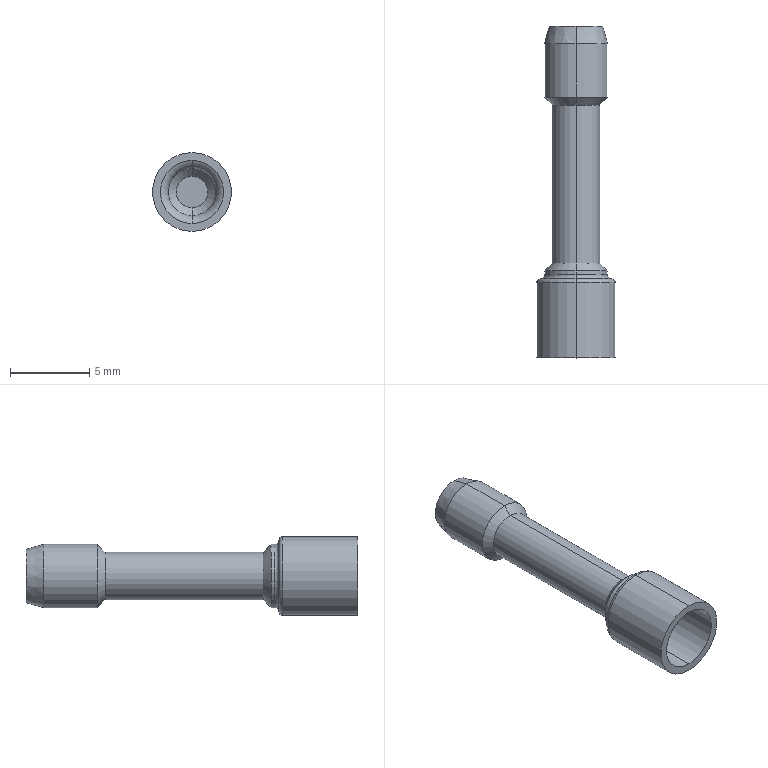Component | SolidWorks | PenTail-1 | 1 solid | 37 faces | box 5 x 21 x 5 mm | volume 112 mm3 | cylinder 16 | cone 12 | torus 6 | plane 3 | commonest cylinder face diameters 3 x6 4 x6 2 x2 5 x2
STEP:
#1=CARTESIAN_POINT('',(-2.232,1.614,-1.121));
#2=VERTEX_POINT('',#1);
#3=CARTESIAN_POINT('',(-2.232,1.614,-1.239));
#4=VERTEX_POINT('',#3);
#5=CARTESIAN_POINT('',(-2.232,1.614,-1.18));
#6=DIRECTION('',(0.,1.,0.));
#7=DIRECTION('',(0.,0.,-1.));
#8=AXIS2_PLACEMENT_3D('',#5,#6,#7);
#9=CIRCLE('',#8,0.05906);
#10=EDGE_CURVE('',#2,#4,#9,.T.);
#11=ORIENTED_EDGE('',*,*,#10,.T.);
#12=CARTESIAN_POINT('',(-2.232,1.586,-1.258));
#13=VERTEX_POINT('',#12);
#14=CARTESIAN_POINT('',(-2.232,1.614,-1.268));
#15=DIRECTION('',(1.,0.,0.));
#16=DIRECTION('',(0.,0.,-1.));
#17=AXIS2_PLACEMENT_3D('',#14,#15,#16);
#18=CIRCLE('',#17,0.02953);
#19=EDGE_CURVE('',#4,#13,#18,.T.);
#20=ORIENTED_EDGE('',*,*,#19,.T.);
#21=CARTESIAN_POINT('',(-2.232,1.586,-1.101));
#22=VERTEX_POINT('',#21);
#23=CARTESIAN_POINT('',(-2.232,1.586,-1.18));
#24=DIRECTION('',(0.,-1.,0.));
#25=DIRECTION('',(0.,0.,1.));
#26=AXIS2_PLACEMENT_3D('',#23,#24,#25);
#27=CIRCLE('',#26,0.07874);
#28=EDGE_CURVE('',#13,#22,#27,.T.);
#29=ORIENTED_EDGE('',*,*,#28,.T.);
#30=CARTESIAN_POINT('',(-2.232,1.614,-1.091));
#31=DIRECTION('',(-1.,0.,0.));
#32=DIRECTION('',(0.,0.,1.));
#33=AXIS2_PLACEMENT_3D('',#30,#31,#32);
#34=CIRCLE('',#33,0.02953);
#35=EDGE_CURVE('',#2,#22,#34,.T.);
#36=ORIENTED_EDGE('',*,*,#35,.F.);
#37=EDGE_LOOP('',(#11,#20,#29,#36));
#38=FACE_OUTER_BOUND('',#37,.T.);
#39=CARTESIAN_POINT('',(-2.232,1.614,-1.18));
#40=DIRECTION('',(0.,1.,0.));
#41=DIRECTION('',(0.,0.,1.));
#42=AXIS2_PLACEMENT_3D('',#39,#40,#41);
#43=TOROIDAL_SURFACE('',#42,0.08858,0.02953);
#44=ADVANCED_FACE('',(#38),#43,.T.);
#45=CARTESIAN_POINT('',(-2.232,2.214,-1.231));
#46=VERTEX_POINT('',#45);
#47=CARTESIAN_POINT('',(-2.232,2.214,-1.128));
#48=VERTEX_POINT('',#47);
#49=CARTESIAN_POINT('',(-2.232,2.214,-1.18));
#50=DIRECTION('',(0.,1.,0.));
#51=DIRECTION('',(0.,0.,1.));
#52=AXIS2_PLACEMENT_3D('',#49,#50,#51);
#53=CIRCLE('',#52,0.05182);
#54=EDGE_CURVE('',#46,#48,#53,.T.);
#55=ORIENTED_EDGE('',*,*,#54,.T.);
#56=CARTESIAN_POINT('',(-2.232,2.187,-1.121));
#57=VERTEX_POINT('',#56);
#58=CARTESIAN_POINT('',(-2.232,2.185,-1.12));
#59=DIRECTION('',(0.,-0.9659,0.2588));
#60=VECTOR('',#59,39.37);
#61=LINE('',#58,#60);
#62=EDGE_CURVE('',#48,#57,#61,.T.);
#63=ORIENTED_EDGE('',*,*,#62,.T.);
#64=CARTESIAN_POINT('',(-2.232,2.187,-1.239));
#65=VERTEX_POINT('',#64);
#66=CARTESIAN_POINT('',(-2.232,2.187,-1.18));
#67=DIRECTION('',(0.,-1.,0.));
#68=DIRECTION('',(0.,0.,-1.));
#69=AXIS2_PLACEMENT_3D('',#66,#67,#68);
#70=CIRCLE('',#69,0.05906);
#71=EDGE_CURVE('',#57,#65,#70,.T.);
#72=ORIENTED_EDGE('',*,*,#71,.T.);
#73=CARTESIAN_POINT('',(-2.232,2.185,-1.239));
#74=DIRECTION('',(0.,-0.9659,-0.2588));
#75=VECTOR('',#74,39.37);
#76=LINE('',#73,#75);
#77=EDGE_CURVE('',#46,#65,#76,.T.);
#78=ORIENTED_EDGE('',*,*,#77,.F.);
#79=EDGE_LOOP('',(#55,#63,#72,#78));
#80=FACE_OUTER_BOUND('',#79,.T.);
#81=CARTESIAN_POINT('',(-2.232,2.185,-1.18));
#82=DIRECTION('',(0.,-1.,0.));
#83=DIRECTION('',(0.,0.,-1.));
#84=AXIS2_PLACEMENT_3D('',#81,#82,#83);
#85=CONICAL_SURFACE('',#84,0.05973,0.2618);
#86=ADVANCED_FACE('',(#80),#85,.F.);
#87=CARTESIAN_POINT('',(-2.232,1.635,-1.14));
#88=VERTEX_POINT('',#87);
#89=CARTESIAN_POINT('',(-2.232,1.635,-1.219));
#90=VERTEX_POINT('',#89);
#91=CARTESIAN_POINT('',(-2.232,1.635,-1.18));
#92=DIRECTION('',(0.,-1.,0.));
#93=DIRECTION('',(0.,0.,-1.));
#94=AXIS2_PLACEMENT_3D('',#91,#92,#93);
#95=CIRCLE('',#94,0.03937);
#96=EDGE_CURVE('',#88,#90,#95,.T.);
#97=ORIENTED_EDGE('',*,*,#96,.F.);
#98=CARTESIAN_POINT('',(-2.232,1.615,-1.121));
#99=VERTEX_POINT('',#98);
#100=CARTESIAN_POINT('',(-2.232,1.61,-1.115));
#101=DIRECTION('',(0.,-0.7071,0.7071));
#102=VECTOR('',#101,39.37);
#103=LINE('',#100,#102);
#104=EDGE_CURVE('',#88,#99,#103,.T.);
#105=ORIENTED_EDGE('',*,*,#104,.T.);
#106=CARTESIAN_POINT('',(-2.232,1.615,-1.239));
#107=VERTEX_POINT('',#106);
#108=CARTESIAN_POINT('',(-2.232,1.615,-1.18));
#109=DIRECTION('',(0.,-1.,0.));
#110=DIRECTION('',(0.,0.,-1.));
#111=AXIS2_PLACEMENT_3D('',#108,#109,#110);
#112=CIRCLE('',#111,0.05906);
#113=EDGE_CURVE('',#99,#107,#112,.T.);
#114=ORIENTED_EDGE('',*,*,#113,.T.);
#115=CARTESIAN_POINT('',(-2.232,1.61,-1.244));
#116=DIRECTION('',(0.,-0.7071,-0.7071));
#117=VECTOR('',#116,39.37);
#118=LINE('',#115,#117);
#119=EDGE_CURVE('',#90,#107,#118,.T.);
#120=ORIENTED_EDGE('',*,*,#119,.F.);
#121=EDGE_LOOP('',(#97,#105,#114,#120));
#122=FACE_OUTER_BOUND('',#121,.T.);
#123=CARTESIAN_POINT('',(-2.232,1.61,-1.18));
#124=DIRECTION('',(0.,-1.,0.));
#125=DIRECTION('',(0.,0.,-1.));
#126=AXIS2_PLACEMENT_3D('',#123,#124,#125);
#127=CONICAL_SURFACE('',#126,0.06482,0.7854);
#128=ADVANCED_FACE('',(#122),#127,.F.);
#129=CARTESIAN_POINT('',(-2.232,2.045,-1.14));
#130=VERTEX_POINT('',#129);
#131=CARTESIAN_POINT('',(-2.232,2.045,-1.219));
#132=VERTEX_POINT('',#131);
#133=CARTESIAN_POINT('',(-2.232,2.045,-1.18));
#134=DIRECTION('',(0.,-1.,0.));
#135=DIRECTION('',(0.,0.,1.));
#136=AXIS2_PLACEMENT_3D('',#133,#134,#135);
#137=CIRCLE('',#136,0.03937);
#138=EDGE_CURVE('',#130,#132,#137,.T.);
#139=ORIENTED_EDGE('',*,*,#138,.T.);
#140=CARTESIAN_POINT('',(-2.232,2.065,-1.239));
#141=VERTEX_POINT('',#140);
#142=CARTESIAN_POINT('',(-2.232,2.051,-1.225));
#143=DIRECTION('',(0.,0.7071,-0.7071));
#144=VECTOR('',#143,39.37);
#145=LINE('',#142,#144);
#146=EDGE_CURVE('',#132,#141,#145,.T.);
#147=ORIENTED_EDGE('',*,*,#146,.T.);
#148=CARTESIAN_POINT('',(-2.232,2.065,-1.121));
#149=VERTEX_POINT('',#148);
#150=CARTESIAN_POINT('',(-2.232,2.065,-1.18));
#151=DIRECTION('',(0.,1.,0.));
#152=DIRECTION('',(0.,0.,1.));
#153=AXIS2_PLACEMENT_3D('',#150,#151,#152);
#154=CIRCLE('',#153,0.05906);
#155=EDGE_CURVE('',#141,#149,#154,.T.);
#156=ORIENTED_EDGE('',*,*,#155,.T.);
#157=CARTESIAN_POINT('',(-2.232,2.051,-1.134));
#158=DIRECTION('',(0.,0.7071,0.7071));
#159=VECTOR('',#158,39.37);
#160=LINE('',#157,#159);
#161=EDGE_CURVE('',#130,#149,#160,.T.);
#162=ORIENTED_EDGE('',*,*,#161,.F.);
#163=EDGE_LOOP('',(#139,#147,#156,#162));
#164=FACE_OUTER_BOUND('',#163,.T.);
#165=CARTESIAN_POINT('',(-2.232,2.051,-1.18));
#166=DIRECTION('',(0.,1.,0.));
#167=DIRECTION('',(0.,0.,1.));
#168=AXIS2_PLACEMENT_3D('',#165,#166,#167);
#169=CONICAL_SURFACE('',#168,0.04514,0.7854);
#170=ADVANCED_FACE('',(#164),#169,.F.);
#171=ORIENTED_EDGE('',*,*,#71,.F.);
#172=CARTESIAN_POINT('',(-2.232,1.407,-1.121));
#173=DIRECTION('',(0.,-1.,0.));
#174=VECTOR('',#173,39.37);
#175=LINE('',#172,#174);
#176=EDGE_CURVE('',#57,#149,#175,.T.);
#177=ORIENTED_EDGE('',*,*,#176,.T.);
#178=ORIENTED_EDGE('',*,*,#155,.F.);
#179=CARTESIAN_POINT('',(-2.232,1.407,-1.239));
#180=DIRECTION('',(0.,-1.,0.));
#181=VECTOR('',#180,39.37);
#182=LINE('',#179,#181);
#183=EDGE_CURVE('',#65,#141,#182,.T.);
#184=ORIENTED_EDGE('',*,*,#183,.F.);
#185=EDGE_LOOP('',(#171,#177,#178,#184));
#186=FACE_OUTER_BOUND('',#185,.T.);
#187=CARTESIAN_POINT('',(-2.232,1.407,-1.18));
#188=DIRECTION('',(0.,-1.,0.));
#189=DIRECTION('',(0.,0.,-1.));
#190=AXIS2_PLACEMENT_3D('',#187,#188,#189);
#191=CYLINDRICAL_SURFACE('',#190,0.05906);
#192=ADVANCED_FACE('',(#186),#191,.F.);
#193=ORIENTED_EDGE('',*,*,#138,.F.);
#194=CARTESIAN_POINT('',(-2.232,1.407,-1.14));
#195=DIRECTION('',(0.,-1.,0.));
#196=VECTOR('',#195,39.37);
#197=LINE('',#194,#196);
#198=EDGE_CURVE('',#130,#88,#197,.T.);
#199=ORIENTED_EDGE('',*,*,#198,.T.);
#200=ORIENTED_EDGE('',*,*,#96,.T.);
#201=CARTESIAN_POINT('',(-2.232,1.407,-1.219));
#202=DIRECTION('',(0.,-1.,0.));
#203=VECTOR('',#202,39.37);
#204=LINE('',#201,#203);
#205=EDGE_CURVE('',#132,#90,#204,.T.);
#206=ORIENTED_EDGE('',*,*,#205,.F.);
#207=EDGE_LOOP('',(#193,#199,#200,#206));
#208=FACE_OUTER_BOUND('',#207,.T.);
#209=CARTESIAN_POINT('',(-2.232,1.407,-1.18));
#210=DIRECTION('',(0.,-1.,0.));
#211=DIRECTION('',(0.,0.,-1.));
#212=AXIS2_PLACEMENT_3D('',#209,#210,#211);
#213=CYLINDRICAL_SURFACE('',#212,0.03937);
#214=ADVANCED_FACE('',(#208),#213,.F.);
#215=ORIENTED_EDGE('',*,*,#113,.F.);
#216=CARTESIAN_POINT('',(-2.232,1.407,-1.121));
#217=DIRECTION('',(0.,-1.,0.));
#218=VECTOR('',#217,39.37);
#219=LINE('',#216,#218);
#220=EDGE_CURVE('',#99,#2,#219,.T.);
#221=ORIENTED_EDGE('',*,*,#220,.T.);
#222=CARTESIAN_POINT('',(-2.232,1.614,-1.18));
#223=DIRECTION('',(0.,1.,0.));
#224=DIRECTION('',(0.,0.,-1.));
#225=AXIS2_PLACEMENT_3D('',#222,#223,#224);
#226=CIRCLE('',#225,0.05906);
#227=EDGE_CURVE('',#4,#2,#226,.T.);
#228=ORIENTED_EDGE('',*,*,#227,.F.);
#229=CARTESIAN_POINT('',(-2.232,1.407,-1.239));
#230=DIRECTION('',(0.,-1.,0.));
#231=VECTOR('',#230,39.37);
#232=LINE('',#229,#231);
#233=EDGE_CURVE('',#107,#4,#232,.T.);
#234=ORIENTED_EDGE('',*,*,#233,.F.);
#235=EDGE_LOOP('',(#215,#221,#228,#234));
#236=FACE_OUTER_BOUND('',#235,.T.);
#237=CARTESIAN_POINT('',(-2.232,1.407,-1.18));
#238=DIRECTION('',(0.,-1.,0.));
#239=DIRECTION('',(0.,0.,-1.));
#240=AXIS2_PLACEMENT_3D('',#237,#238,#239);
#241=CYLINDRICAL_SURFACE('',#240,0.05906);
#242=ADVANCED_FACE('',(#236),#241,.F.);
#243=CARTESIAN_POINT('',(-2.232,1.586,-1.18));
#244=DIRECTION('',(0.,-1.,0.));
#245=DIRECTION('',(0.,0.,1.));
#246=AXIS2_PLACEMENT_3D('',#243,#244,#245);
#247=CIRCLE('',#246,0.07874);
#248=EDGE_CURVE('',#22,#13,#247,.T.);
#249=ORIENTED_EDGE('',*,*,#248,.F.);
#250=CARTESIAN_POINT('',(-2.232,1.407,-1.101));
#251=VERTEX_POINT('',#250);
#252=CARTESIAN_POINT('',(-2.232,1.407,-1.101));
#253=DIRECTION('',(0.,-1.,0.));
#254=VECTOR('',#253,39.37);
#255=LINE('',#252,#254);
#256=EDGE_CURVE('',#22,#251,#255,.T.);
#257=ORIENTED_EDGE('',*,*,#256,.T.);
#258=CARTESIAN_POINT('',(-2.232,1.407,-1.258));
#259=VERTEX_POINT('',#258);
#260=CARTESIAN_POINT('',(-2.232,1.407,-1.18));
#261=DIRECTION('',(0.,-1.,0.));
#262=DIRECTION('',(0.,0.,-1.));
#263=AXIS2_PLACEMENT_3D('',#260,#261,#262);
#264=CIRCLE('',#263,0.07874);
#265=EDGE_CURVE('',#251,#259,#264,.T.);
#266=ORIENTED_EDGE('',*,*,#265,.T.);
#267=CARTESIAN_POINT('',(-2.232,1.407,-1.258));
#268=DIRECTION('',(0.,-1.,0.));
#269=VECTOR('',#268,39.37);
#270=LINE('',#267,#269);
#271=EDGE_CURVE('',#13,#259,#270,.T.);
#272=ORIENTED_EDGE('',*,*,#271,.F.);
#273=EDGE_LOOP('',(#249,#257,#266,#272));
#274=FACE_OUTER_BOUND('',#273,.T.);
#275=CARTESIAN_POINT('',(-2.232,1.407,-1.18));
#276=DIRECTION('',(0.,-1.,0.));
#277=DIRECTION('',(0.,0.,-1.));
#278=AXIS2_PLACEMENT_3D('',#275,#276,#277);
#279=CYLINDRICAL_SURFACE('',#278,0.07874);
#280=ADVANCED_FACE('',(#274),#279,.F.);
#281=CARTESIAN_POINT('',(-2.232,1.594,-1.278));
#282=VERTEX_POINT('',#281);
#283=CARTESIAN_POINT('',(-2.232,1.594,-1.081));
#284=VERTEX_POINT('',#283);
#285=CARTESIAN_POINT('',(-2.232,1.594,-1.18));
#286=DIRECTION('',(0.,-1.,0.));
#287=DIRECTION('',(0.,0.,1.));
#288=AXIS2_PLACEMENT_3D('',#285,#286,#287);
#289=CIRCLE('',#288,0.09843);
#290=EDGE_CURVE('',#282,#284,#289,.T.);
#291=ORIENTED_EDGE('',*,*,#290,.F.);
#292=CARTESIAN_POINT('',(-2.232,1.604,-1.268));
#293=VERTEX_POINT('',#292);
#294=CARTESIAN_POINT('',(-2.232,1.594,-1.268));
#295=DIRECTION('',(1.,0.,0.));
#296=DIRECTION('',(0.,0.,-1.));
#297=AXIS2_PLACEMENT_3D('',#294,#295,#296);
#298=CIRCLE('',#297,0.009843);
#299=EDGE_CURVE('',#282,#293,#298,.T.);
#300=ORIENTED_EDGE('',*,*,#299,.T.);
#301=CARTESIAN_POINT('',(-2.232,1.604,-1.091));
#302=VERTEX_POINT('',#301);
#303=CARTESIAN_POINT('',(-2.232,1.604,-1.18));
#304=DIRECTION('',(0.,-1.,0.));
#305=DIRECTION('',(0.,0.,1.));
#306=AXIS2_PLACEMENT_3D('',#303,#304,#305);
#307=CIRCLE('',#306,0.08858);
#308=EDGE_CURVE('',#293,#302,#307,.T.);
#309=ORIENTED_EDGE('',*,*,#308,.T.);
#310=CARTESIAN_POINT('',(-2.232,1.594,-1.091));
#311=DIRECTION('',(-1.,0.,0.));
#312=DIRECTION('',(0.,0.,1.));
#313=AXIS2_PLACEMENT_3D('',#310,#311,#312);
#314=CIRCLE('',#313,0.009843);
#315=EDGE_CURVE('',#284,#302,#314,.T.);
#316=ORIENTED_EDGE('',*,*,#315,.F.);
#317=EDGE_LOOP('',(#291,#300,#309,#316));
#318=FACE_OUTER_BOUND('',#317,.T.);
#319=CARTESIAN_POINT('',(-2.232,1.594,-1.18));
#320=DIRECTION('',(0.,1.,0.));
#321=DIRECTION('',(0.,0.,1.));
#322=AXIS2_PLACEMENT_3D('',#319,#320,#321);
#323=TOROIDAL_SURFACE('',#322,0.08858,0.009843);
#324=ADVANCED_FACE('',(#318),#323,.T.);
#325=CARTESIAN_POINT('',(-2.232,1.614,-1.258));
#326=VERTEX_POINT('',#325);
#327=CARTESIAN_POINT('',(-2.232,1.614,-1.101));
#328=VERTEX_POINT('',#327);
#329=CARTESIAN_POINT('',(-2.232,1.614,-1.18));
#330=DIRECTION('',(0.,1.,0.));
#331=DIRECTION('',(0.,0.,1.));
#332=AXIS2_PLACEMENT_3D('',#329,#330,#331);
#333=CIRCLE('',#332,0.07874);
#334=EDGE_CURVE('',#326,#328,#333,.T.);
#335=ORIENTED_EDGE('',*,*,#334,.F.);
#336=CARTESIAN_POINT('',(-2.232,1.614,-1.268));
#337=DIRECTION('',(1.,0.,0.));
#338=DIRECTION('',(0.,0.,-1.));
#339=AXIS2_PLACEMENT_3D('',#336,#337,#338);
#340=CIRCLE('',#339,0.009843);
#341=EDGE_CURVE('',#326,#293,#340,.T.);
#342=ORIENTED_EDGE('',*,*,#341,.T.);
#343=CARTESIAN_POINT('',(-2.232,1.604,-1.18));
#344=DIRECTION('',(0.,-1.,0.));
#345=DIRECTION('',(0.,0.,1.));
#346=AXIS2_PLACEMENT_3D('',#343,#344,#345);
#347=CIRCLE('',#346,0.08858);
#348=EDGE_CURVE('',#302,#293,#347,.T.);
#349=ORIENTED_EDGE('',*,*,#348,.F.);
#350=CARTESIAN_POINT('',(-2.232,1.614,-1.091));
#351=DIRECTION('',(-1.,0.,0.));
#352=DIRECTION('',(0.,0.,1.));
#353=AXIS2_PLACEMENT_3D('',#350,#351,#352);
#354=CIRCLE('',#353,0.009843);
#355=EDGE_CURVE('',#328,#302,#354,.T.);
#356=ORIENTED_EDGE('',*,*,#355,.F.);
#357=EDGE_LOOP('',(#335,#342,#349,#356));
#358=FACE_OUTER_BOUND('',#357,.T.);
#359=CARTESIAN_POINT('',(-2.232,1.614,-1.18));
#360=DIRECTION('',(0.,1.,0.));
#361=DIRECTION('',(0.,0.,1.));
#362=AXIS2_PLACEMENT_3D('',#359,#360,#361);
#363=TOROIDAL_SURFACE('',#362,0.08858,0.009843);
#364=ADVANCED_FACE('',(#358),#363,.F.);
#365=CARTESIAN_POINT('',(-2.232,2.234,-1.113));
#366=VERTEX_POINT('',#365);
#367=CARTESIAN_POINT('',(-2.232,2.234,-1.247));
#368=VERTEX_POINT('',#367);
#369=CARTESIAN_POINT('',(-2.232,2.234,-1.18));
#370=DIRECTION('',(0.,1.,0.));
#371=DIRECTION('',(0.,0.,1.));
#372=AXIS2_PLACEMENT_3D('',#369,#370,#371);
#373=CIRCLE('',#372,0.06693);
#374=EDGE_CURVE('',#366,#368,#373,.T.);
#375=ORIENTED_EDGE('',*,*,#374,.F.);
#376=CARTESIAN_POINT('',(-2.232,2.19,-1.101));
#377=VERTEX_POINT('',#376);
#378=CARTESIAN_POINT('',(-2.232,2.19,-1.101));
#379=DIRECTION('',(0.,-0.9659,0.2588));
#380=VECTOR('',#379,39.37);
#381=LINE('',#378,#380);
#382=EDGE_CURVE('',#366,#377,#381,.T.);
#383=ORIENTED_EDGE('',*,*,#382,.T.);
#384=CARTESIAN_POINT('',(-2.232,2.19,-1.258));
#385=VERTEX_POINT('',#384);
#386=CARTESIAN_POINT('',(-2.232,2.19,-1.18));
#387=DIRECTION('',(0.,-1.,0.));
#388=DIRECTION('',(0.,0.,1.));
#389=AXIS2_PLACEMENT_3D('',#386,#387,#388);
#390=CIRCLE('',#389,0.07874);
#391=EDGE_CURVE('',#385,#377,#390,.T.);
#392=ORIENTED_EDGE('',*,*,#391,.F.);
#393=CARTESIAN_POINT('',(-2.232,2.19,-1.258));
#394=DIRECTION('',(0.,-0.9659,-0.2588));
#395=VECTOR('',#394,39.37);
#396=LINE('',#393,#395);
#397=EDGE_CURVE('',#368,#385,#396,.T.);
#398=ORIENTED_EDGE('',*,*,#397,.F.);
#399=EDGE_LOOP('',(#375,#383,#392,#398));
#400=FACE_OUTER_BOUND('',#399,.T.);
#401=CARTESIAN_POINT('',(-2.232,2.19,-1.18));
#402=DIRECTION('',(0.,-1.,0.));
#403=DIRECTION('',(0.,0.,-1.));
#404=AXIS2_PLACEMENT_3D('',#401,#402,#403);
#405=CONICAL_SURFACE('',#404,0.07874,0.2618);
#406=ADVANCED_FACE('',(#400),#405,.T.);
#407=CARTESIAN_POINT('',(-2.232,1.643,-1.239));
#408=VERTEX_POINT('',#407);
#409=CARTESIAN_POINT('',(-2.232,1.643,-1.121));
#410=VERTEX_POINT('',#409);
#411=CARTESIAN_POINT('',(-2.232,1.643,-1.18));
#412=DIRECTION('',(0.,-1.,0.));
#413=DIRECTION('',(0.,0.,-1.));
#414=AXIS2_PLACEMENT_3D('',#411,#412,#413);
#415=CIRCLE('',#414,0.05906);
#416=EDGE_CURVE('',#408,#410,#415,.T.);
#417=ORIENTED_EDGE('',*,*,#416,.T.);
#418=CARTESIAN_POINT('',(-2.232,1.623,-1.101));
#419=VERTEX_POINT('',#418);
#420=CARTESIAN_POINT('',(-2.232,1.623,-1.101));
#421=DIRECTION('',(0.,-0.7071,0.7071));
#422=VECTOR('',#421,39.37);
#423=LINE('',#420,#422);
#424=EDGE_CURVE('',#410,#419,#423,.T.);
#425=ORIENTED_EDGE('',*,*,#424,.T.);
#426=CARTESIAN_POINT('',(-2.232,1.623,-1.258));
#427=VERTEX_POINT('',#426);
#428=CARTESIAN_POINT('',(-2.232,1.623,-1.18));
#429=DIRECTION('',(0.,-1.,0.));
#430=DIRECTION('',(0.,0.,1.));
#431=AXIS2_PLACEMENT_3D('',#428,#429,#430);
#432=CIRCLE('',#431,0.07874);
#433=EDGE_CURVE('',#427,#419,#432,.T.);
#434=ORIENTED_EDGE('',*,*,#433,.F.);
#435=CARTESIAN_POINT('',(-2.232,1.623,-1.258));
#436=DIRECTION('',(0.,-0.7071,-0.7071));
#437=VECTOR('',#436,39.37);
#438=LINE('',#435,#437);
#439=EDGE_CURVE('',#408,#427,#438,.T.);
#440=ORIENTED_EDGE('',*,*,#439,.F.);
#441=EDGE_LOOP('',(#417,#425,#434,#440));
#442=FACE_OUTER_BOUND('',#441,.T.);
#443=CARTESIAN_POINT('',(-2.232,1.623,-1.18));
#444=DIRECTION('',(0.,-1.,0.));
#445=DIRECTION('',(0.,0.,-1.));
#446=AXIS2_PLACEMENT_3D('',#443,#444,#445);
#447=CONICAL_SURFACE('',#446,0.07874,0.7854);
#448=ADVANCED_FACE('',(#442),#447,.T.);
#449=CARTESIAN_POINT('',(-2.232,2.037,-1.239));
#450=VERTEX_POINT('',#449);
#451=CARTESIAN_POINT('',(-2.232,2.037,-1.121));
#452=VERTEX_POINT('',#451);
#453=CARTESIAN_POINT('',(-2.232,2.037,-1.18));
#454=DIRECTION('',(0.,-1.,0.));
#455=DIRECTION('',(0.,0.,-1.));
#456=AXIS2_PLACEMENT_3D('',#453,#454,#455);
#457=CIRCLE('',#456,0.05906);
#458=EDGE_CURVE('',#450,#452,#457,.T.);
#459=ORIENTED_EDGE('',*,*,#458,.F.);
#460=CARTESIAN_POINT('',(-2.232,2.057,-1.258));
#461=VERTEX_POINT('',#460);
#462=CARTESIAN_POINT('',(-2.232,2.037,-1.239));
#463=DIRECTION('',(0.,0.7071,-0.7071));
#464=VECTOR('',#463,39.37);
#465=LINE('',#462,#464);
#466=EDGE_CURVE('',#450,#461,#465,.T.);
#467=ORIENTED_EDGE('',*,*,#466,.T.);
#468=CARTESIAN_POINT('',(-2.232,2.057,-1.101));
#469=VERTEX_POINT('',#468);
#470=CARTESIAN_POINT('',(-2.232,2.057,-1.18));
#471=DIRECTION('',(0.,1.,0.));
#472=DIRECTION('',(0.,0.,-1.));
#473=AXIS2_PLACEMENT_3D('',#470,#471,#472);
#474=CIRCLE('',#473,0.07874);
#475=EDGE_CURVE('',#469,#461,#474,.T.);
#476=ORIENTED_EDGE('',*,*,#475,.F.);
#477=CARTESIAN_POINT('',(-2.232,2.037,-1.121));
#478=DIRECTION('',(0.,0.7071,0.7071));
#479=VECTOR('',#478,39.37);
#480=LINE('',#477,#479);
#481=EDGE_CURVE('',#452,#469,#480,.T.);
#482=ORIENTED_EDGE('',*,*,#481,.F.);
#483=EDGE_LOOP('',(#459,#467,#476,#482));
#484=FACE_OUTER_BOUND('',#483,.T.);
#485=CARTESIAN_POINT('',(-2.232,2.037,-1.18));
#486=DIRECTION('',(0.,1.,0.));
#487=DIRECTION('',(0.,0.,1.));
#488=AXIS2_PLACEMENT_3D('',#485,#486,#487);
#489=CONICAL_SURFACE('',#488,0.05906,0.7854);
#490=ADVANCED_FACE('',(#484),#489,.T.);
#491=ORIENTED_EDGE('',*,*,#391,.T.);
#492=CARTESIAN_POINT('',(-2.232,1.407,-1.101));
#493=DIRECTION('',(0.,-1.,0.));
#494=VECTOR('',#493,39.37);
#495=LINE('',#492,#494);
#496=EDGE_CURVE('',#377,#469,#495,.T.);
#497=ORIENTED_EDGE('',*,*,#496,.T.);
#498=ORIENTED_EDGE('',*,*,#475,.T.);
#499=CARTESIAN_POINT('',(-2.232,1.407,-1.258));
#500=DIRECTION('',(0.,-1.,0.));
#501=VECTOR('',#500,39.37);
#502=LINE('',#499,#501);
#503=EDGE_CURVE('',#385,#461,#502,.T.);
#504=ORIENTED_EDGE('',*,*,#503,.F.);
#505=EDGE_LOOP('',(#491,#497,#498,#504));
#506=FACE_OUTER_BOUND('',#505,.T.);
#507=CARTESIAN_POINT('',(-2.232,1.407,-1.18));
#508=DIRECTION('',(0.,-1.,0.));
#509=DIRECTION('',(0.,0.,-1.));
#510=AXIS2_PLACEMENT_3D('',#507,#508,#509);
#511=CYLINDRICAL_SURFACE('',#510,0.07874);
#512=ADVANCED_FACE('',(#506),#511,.T.);
#513=ORIENTED_EDGE('',*,*,#458,.T.);
#514=CARTESIAN_POINT('',(-2.232,1.407,-1.121));
#515=DIRECTION('',(0.,-1.,0.));
#516=VECTOR('',#515,39.37);
#517=LINE('',#514,#516);
#518=EDGE_CURVE('',#452,#410,#517,.T.);
#519=ORIENTED_EDGE('',*,*,#518,.T.);
#520=ORIENTED_EDGE('',*,*,#416,.F.);
#521=CARTESIAN_POINT('',(-2.232,1.407,-1.239));
#522=DIRECTION('',(0.,-1.,0.));
#523=VECTOR('',#522,39.37);
#524=LINE('',#521,#523);
#525=EDGE_CURVE('',#450,#408,#524,.T.);
#526=ORIENTED_EDGE('',*,*,#525,.F.);
#527=EDGE_LOOP('',(#513,#519,#520,#526));
#528=FACE_OUTER_BOUND('',#527,.T.);
#529=CARTESIAN_POINT('',(-2.232,1.407,-1.18));
#530=DIRECTION('',(0.,-1.,0.));
#531=DIRECTION('',(0.,0.,-1.));
#532=AXIS2_PLACEMENT_3D('',#529,#530,#531);
#533=CYLINDRICAL_SURFACE('',#532,0.05906);
#534=ADVANCED_FACE('',(#528),#533,.T.);
#535=ORIENTED_EDGE('',*,*,#433,.T.);
#536=CARTESIAN_POINT('',(-2.232,1.407,-1.101));
#537=DIRECTION('',(0.,-1.,0.));
#538=VECTOR('',#537,39.37);
#539=LINE('',#536,#538);
#540=EDGE_CURVE('',#419,#328,#539,.T.);
#541=ORIENTED_EDGE('',*,*,#540,.T.);
#542=CARTESIAN_POINT('',(-2.232,1.614,-1.18));
#543=DIRECTION('',(0.,1.,0.));
#544=DIRECTION('',(0.,0.,1.));
#545=AXIS2_PLACEMENT_3D('',#542,#543,#544);
#546=CIRCLE('',#545,0.07874);
#547=EDGE_CURVE('',#328,#326,#546,.T.);
#548=ORIENTED_EDGE('',*,*,#547,.T.);
#549=CARTESIAN_POINT('',(-2.232,1.407,-1.258));
#550=DIRECTION('',(0.,-1.,0.));
#551=VECTOR('',#550,39.37);
#552=LINE('',#549,#551);
#553=EDGE_CURVE('',#427,#326,#552,.T.);
#554=ORIENTED_EDGE('',*,*,#553,.F.);
#555=EDGE_LOOP('',(#535,#541,#548,#554));
#556=FACE_OUTER_BOUND('',#555,.T.);
#557=CARTESIAN_POINT('',(-2.232,1.407,-1.18));
#558=DIRECTION('',(0.,-1.,0.));
#559=DIRECTION('',(0.,0.,-1.));
#560=AXIS2_PLACEMENT_3D('',#557,#558,#559);
#561=CYLINDRICAL_SURFACE('',#560,0.07874);
#562=ADVANCED_FACE('',(#556),#561,.T.);
#563=ORIENTED_EDGE('',*,*,#290,.T.);
#564=CARTESIAN_POINT('',(-2.232,1.407,-1.081));
#565=VERTEX_POINT('',#564);
#566=CARTESIAN_POINT('',(-2.232,1.407,-1.081));
#567=DIRECTION('',(0.,-1.,0.));
#568=VECTOR('',#567,39.37);
#569=LINE('',#566,#568);
#570=EDGE_CURVE('',#284,#565,#569,.T.);
#571=ORIENTED_EDGE('',*,*,#570,.T.);
#572=CARTESIAN_POINT('',(-2.232,1.407,-1.278));
#573=VERTEX_POINT('',#572);
#574=CARTESIAN_POINT('',(-2.232,1.407,-1.18));
#575=DIRECTION('',(0.,-1.,0.));
#576=DIRECTION('',(0.,0.,-1.));
#577=AXIS2_PLACEMENT_3D('',#574,#575,#576);
#578=CIRCLE('',#577,0.09843);
#579=EDGE_CURVE('',#573,#565,#578,.T.);
#580=ORIENTED_EDGE('',*,*,#579,.F.);
#581=CARTESIAN_POINT('',(-2.232,1.407,-1.278));
#582=DIRECTION('',(0.,-1.,0.));
#583=VECTOR('',#582,39.37);
#584=LINE('',#581,#583);
#585=EDGE_CURVE('',#282,#573,#584,.T.);
#586=ORIENTED_EDGE('',*,*,#585,.F.);
#587=EDGE_LOOP('',(#563,#571,#580,#586));
#588=FACE_OUTER_BOUND('',#587,.T.);
#589=CARTESIAN_POINT('',(-2.232,1.407,-1.18));
#590=DIRECTION('',(0.,-1.,0.));
#591=DIRECTION('',(0.,0.,-1.));
#592=AXIS2_PLACEMENT_3D('',#589,#590,#591);
#593=CYLINDRICAL_SURFACE('',#592,0.09843);
#594=ADVANCED_FACE('',(#588),#593,.T.);
#595=CARTESIAN_POINT('',(-2.232,1.407,-1.18));
#596=DIRECTION('',(0.,-1.,0.));
#597=DIRECTION('',(0.,0.,-1.));
#598=AXIS2_PLACEMENT_3D('',#595,#596,#597);
#599=CIRCLE('',#598,0.07874);
#600=EDGE_CURVE('',#259,#251,#599,.T.);
#601=ORIENTED_EDGE('',*,*,#600,.F.);
#602=ORIENTED_EDGE('',*,*,#265,.F.);
#603=EDGE_LOOP('',(#601,#602));
#604=FACE_BOUND('',#603,.T.);
#605=ORIENTED_EDGE('',*,*,#579,.T.);
#606=CARTESIAN_POINT('',(-2.232,1.407,-1.18));
#607=DIRECTION('',(0.,-1.,0.));
#608=DIRECTION('',(0.,0.,-1.));
#609=AXIS2_PLACEMENT_3D('',#606,#607,#608);
#610=CIRCLE('',#609,0.09843);
#611=EDGE_CURVE('',#565,#573,#610,.T.);
#612=ORIENTED_EDGE('',*,*,#611,.T.);
#613=EDGE_LOOP('',(#605,#612));
#614=FACE_OUTER_BOUND('',#613,.T.);
#615=CARTESIAN_POINT('',(-2.232,1.407,-1.18));
#616=DIRECTION('',(0.,-1.,0.));
#617=DIRECTION('',(0.,0.,-1.));
#618=AXIS2_PLACEMENT_3D('',#615,#616,#617);
#619=PLANE('',#618);
#620=ADVANCED_FACE('',(#604,#614),#619,.T.);
#621=ORIENTED_EDGE('',*,*,#570,.F.);
#622=CARTESIAN_POINT('',(-2.232,1.594,-1.18));
#623=DIRECTION('',(0.,-1.,0.));
#624=DIRECTION('',(0.,0.,1.));
#625=AXIS2_PLACEMENT_3D('',#622,#623,#624);
#626=CIRCLE('',#625,0.09843);
#627=EDGE_CURVE('',#284,#282,#626,.T.);
#628=ORIENTED_EDGE('',*,*,#627,.T.);
#629=ORIENTED_EDGE('',*,*,#585,.T.);
#630=ORIENTED_EDGE('',*,*,#611,.F.);
#631=EDGE_LOOP('',(#621,#628,#629,#630));
#632=FACE_OUTER_BOUND('',#631,.T.);
#633=CARTESIAN_POINT('',(-2.232,1.407,-1.18));
#634=DIRECTION('',(0.,-1.,0.));
#635=DIRECTION('',(0.,0.,-1.));
#636=AXIS2_PLACEMENT_3D('',#633,#634,#635);
#637=CYLINDRICAL_SURFACE('',#636,0.09843);
#638=ADVANCED_FACE('',(#632),#637,.T.);
#639=ORIENTED_EDGE('',*,*,#540,.F.);
#640=CARTESIAN_POINT('',(-2.232,1.623,-1.18));
#641=DIRECTION('',(0.,-1.,0.));
#642=DIRECTION('',(0.,0.,1.));
#643=AXIS2_PLACEMENT_3D('',#640,#641,#642);
#644=CIRCLE('',#643,0.07874);
#645=EDGE_CURVE('',#419,#427,#644,.T.);
#646=ORIENTED_EDGE('',*,*,#645,.T.);
#647=ORIENTED_EDGE('',*,*,#553,.T.);
#648=ORIENTED_EDGE('',*,*,#334,.T.);
#649=EDGE_LOOP('',(#639,#646,#647,#648));
#650=FACE_OUTER_BOUND('',#649,.T.);
#651=CARTESIAN_POINT('',(-2.232,1.407,-1.18));
#652=DIRECTION('',(0.,-1.,0.));
#653=DIRECTION('',(0.,0.,-1.));
#654=AXIS2_PLACEMENT_3D('',#651,#652,#653);
#655=CYLINDRICAL_SURFACE('',#654,0.07874);
#656=ADVANCED_FACE('',(#650),#655,.T.);
#657=ORIENTED_EDGE('',*,*,#518,.F.);
#658=CARTESIAN_POINT('',(-2.232,2.037,-1.18));
#659=DIRECTION('',(0.,-1.,0.));
#660=DIRECTION('',(0.,0.,-1.));
#661=AXIS2_PLACEMENT_3D('',#658,#659,#660);
#662=CIRCLE('',#661,0.05906);
#663=EDGE_CURVE('',#452,#450,#662,.T.);
#664=ORIENTED_EDGE('',*,*,#663,.T.);
#665=ORIENTED_EDGE('',*,*,#525,.T.);
#666=CARTESIAN_POINT('',(-2.232,1.643,-1.18));
#667=DIRECTION('',(0.,-1.,0.));
#668=DIRECTION('',(0.,0.,-1.));
#669=AXIS2_PLACEMENT_3D('',#666,#667,#668);
#670=CIRCLE('',#669,0.05906);
#671=EDGE_CURVE('',#410,#408,#670,.T.);
#672=ORIENTED_EDGE('',*,*,#671,.F.);
#673=EDGE_LOOP('',(#657,#664,#665,#672));
#674=FACE_OUTER_BOUND('',#673,.T.);
#675=CARTESIAN_POINT('',(-2.232,1.407,-1.18));
#676=DIRECTION('',(0.,-1.,0.));
#677=DIRECTION('',(0.,0.,-1.));
#678=AXIS2_PLACEMENT_3D('',#675,#676,#677);
#679=CYLINDRICAL_SURFACE('',#678,0.05906);
#680=ADVANCED_FACE('',(#674),#679,.T.);
#681=ORIENTED_EDGE('',*,*,#496,.F.);
#682=CARTESIAN_POINT('',(-2.232,2.19,-1.18));
#683=DIRECTION('',(0.,-1.,0.));
#684=DIRECTION('',(0.,0.,1.));
#685=AXIS2_PLACEMENT_3D('',#682,#683,#684);
#686=CIRCLE('',#685,0.07874);
#687=EDGE_CURVE('',#377,#385,#686,.T.);
#688=ORIENTED_EDGE('',*,*,#687,.T.);
#689=ORIENTED_EDGE('',*,*,#503,.T.);
#690=CARTESIAN_POINT('',(-2.232,2.057,-1.18));
#691=DIRECTION('',(0.,1.,0.));
#692=DIRECTION('',(0.,0.,-1.));
#693=AXIS2_PLACEMENT_3D('',#690,#691,#692);
#694=CIRCLE('',#693,0.07874);
#695=EDGE_CURVE('',#461,#469,#694,.T.);
#696=ORIENTED_EDGE('',*,*,#695,.T.);
#697=EDGE_LOOP('',(#681,#688,#689,#696));
#698=FACE_OUTER_BOUND('',#697,.T.);
#699=CARTESIAN_POINT('',(-2.232,1.407,-1.18));
#700=DIRECTION('',(0.,-1.,0.));
#701=DIRECTION('',(0.,0.,-1.));
#702=AXIS2_PLACEMENT_3D('',#699,#700,#701);
#703=CYLINDRICAL_SURFACE('',#702,0.07874);
#704=ADVANCED_FACE('',(#698),#703,.T.);
#705=CARTESIAN_POINT('',(-2.232,2.234,-1.18));
#706=DIRECTION('',(0.,1.,0.));
#707=DIRECTION('',(0.,0.,1.));
#708=AXIS2_PLACEMENT_3D('',#705,#706,#707);
#709=CIRCLE('',#708,0.06693);
#710=EDGE_CURVE('',#368,#366,#709,.T.);
#711=ORIENTED_EDGE('',*,*,#710,.T.);
#712=ORIENTED_EDGE('',*,*,#374,.T.);
#713=EDGE_LOOP('',(#711,#712));
#714=FACE_OUTER_BOUND('',#713,.T.);
#715=CARTESIAN_POINT('',(-2.232,2.234,-1.258));
#716=DIRECTION('',(0.,1.,0.));
#717=DIRECTION('',(0.,0.,1.));
#718=AXIS2_PLACEMENT_3D('',#715,#716,#717);
#719=PLANE('',#718);
#720=ADVANCED_FACE('',(#714),#719,.T.);
#721=ORIENTED_EDGE('',*,*,#466,.F.);
#722=ORIENTED_EDGE('',*,*,#663,.F.);
#723=ORIENTED_EDGE('',*,*,#481,.T.);
#724=ORIENTED_EDGE('',*,*,#695,.F.);
#725=EDGE_LOOP('',(#721,#722,#723,#724));
#726=FACE_OUTER_BOUND('',#725,.T.);
#727=CARTESIAN_POINT('',(-2.232,2.037,-1.18));
#728=DIRECTION('',(0.,1.,0.));
#729=DIRECTION('',(0.,0.,1.));
#730=AXIS2_PLACEMENT_3D('',#727,#728,#729);
#731=CONICAL_SURFACE('',#730,0.05906,0.7854);
#732=ADVANCED_FACE('',(#726),#731,.T.);
#733=ORIENTED_EDGE('',*,*,#424,.F.);
#734=ORIENTED_EDGE('',*,*,#671,.T.);
#735=ORIENTED_EDGE('',*,*,#439,.T.);
#736=ORIENTED_EDGE('',*,*,#645,.F.);
#737=EDGE_LOOP('',(#733,#734,#735,#736));
#738=FACE_OUTER_BOUND('',#737,.T.);
#739=CARTESIAN_POINT('',(-2.232,1.623,-1.18));
#740=DIRECTION('',(0.,-1.,0.));
#741=DIRECTION('',(0.,0.,-1.));
#742=AXIS2_PLACEMENT_3D('',#739,#740,#741);
#743=CONICAL_SURFACE('',#742,0.07874,0.7854);
#744=ADVANCED_FACE('',(#738),#743,.T.);
#745=ORIENTED_EDGE('',*,*,#382,.F.);
#746=ORIENTED_EDGE('',*,*,#710,.F.);
#747=ORIENTED_EDGE('',*,*,#397,.T.);
#748=ORIENTED_EDGE('',*,*,#687,.F.);
#749=EDGE_LOOP('',(#745,#746,#747,#748));
#750=FACE_OUTER_BOUND('',#749,.T.);
#751=CARTESIAN_POINT('',(-2.232,2.19,-1.18));
#752=DIRECTION('',(0.,-1.,0.));
#753=DIRECTION('',(0.,0.,-1.));
#754=AXIS2_PLACEMENT_3D('',#751,#752,#753);
#755=CONICAL_SURFACE('',#754,0.07874,0.2618);
#756=ADVANCED_FACE('',(#750),#755,.T.);
#757=ORIENTED_EDGE('',*,*,#341,.F.);
#758=ORIENTED_EDGE('',*,*,#547,.F.);
#759=ORIENTED_EDGE('',*,*,#355,.T.);
#760=ORIENTED_EDGE('',*,*,#308,.F.);
#761=EDGE_LOOP('',(#757,#758,#759,#760));
#762=FACE_OUTER_BOUND('',#761,.T.);
#763=CARTESIAN_POINT('',(-2.232,1.614,-1.18));
#764=DIRECTION('',(0.,1.,0.));
#765=DIRECTION('',(0.,0.,1.));
#766=AXIS2_PLACEMENT_3D('',#763,#764,#765);
#767=TOROIDAL_SURFACE('',#766,0.08858,0.009843);
#768=ADVANCED_FACE('',(#762),#767,.F.);
#769=ORIENTED_EDGE('',*,*,#299,.F.);
#770=ORIENTED_EDGE('',*,*,#627,.F.);
#771=ORIENTED_EDGE('',*,*,#315,.T.);
#772=ORIENTED_EDGE('',*,*,#348,.T.);
#773=EDGE_LOOP('',(#769,#770,#771,#772));
#774=FACE_OUTER_BOUND('',#773,.T.);
#775=CARTESIAN_POINT('',(-2.232,1.594,-1.18));
#776=DIRECTION('',(0.,1.,0.));
#777=DIRECTION('',(0.,0.,1.));
#778=AXIS2_PLACEMENT_3D('',#775,#776,#777);
#779=TOROIDAL_SURFACE('',#778,0.08858,0.009843);
#780=ADVANCED_FACE('',(#774),#779,.T.);
#781=ORIENTED_EDGE('',*,*,#256,.F.);
#782=ORIENTED_EDGE('',*,*,#28,.F.);
#783=ORIENTED_EDGE('',*,*,#271,.T.);
#784=ORIENTED_EDGE('',*,*,#600,.T.);
#785=EDGE_LOOP('',(#781,#782,#783,#784));
#786=FACE_OUTER_BOUND('',#785,.T.);
#787=CARTESIAN_POINT('',(-2.232,1.407,-1.18));
#788=DIRECTION('',(0.,-1.,0.));
#789=DIRECTION('',(0.,0.,-1.));
#790=AXIS2_PLACEMENT_3D('',#787,#788,#789);
#791=CYLINDRICAL_SURFACE('',#790,0.07874);
#792=ADVANCED_FACE('',(#786),#791,.F.);
#793=ORIENTED_EDGE('',*,*,#220,.F.);
#794=CARTESIAN_POINT('',(-2.232,1.615,-1.18));
#795=DIRECTION('',(0.,-1.,0.));
#796=DIRECTION('',(0.,0.,-1.));
#797=AXIS2_PLACEMENT_3D('',#794,#795,#796);
#798=CIRCLE('',#797,0.05906);
#799=EDGE_CURVE('',#107,#99,#798,.T.);
#800=ORIENTED_EDGE('',*,*,#799,.F.);
#801=ORIENTED_EDGE('',*,*,#233,.T.);
#802=ORIENTED_EDGE('',*,*,#10,.F.);
#803=EDGE_LOOP('',(#793,#800,#801,#802));
#804=FACE_OUTER_BOUND('',#803,.T.);
#805=CARTESIAN_POINT('',(-2.232,1.407,-1.18));
#806=DIRECTION('',(0.,-1.,0.));
#807=DIRECTION('',(0.,0.,-1.));
#808=AXIS2_PLACEMENT_3D('',#805,#806,#807);
#809=CYLINDRICAL_SURFACE('',#808,0.05906);
#810=ADVANCED_FACE('',(#804),#809,.F.);
#811=ORIENTED_EDGE('',*,*,#198,.F.);
#812=CARTESIAN_POINT('',(-2.232,2.045,-1.18));
#813=DIRECTION('',(0.,-1.,0.));
#814=DIRECTION('',(0.,0.,1.));
#815=AXIS2_PLACEMENT_3D('',#812,#813,#814);
#816=CIRCLE('',#815,0.03937);
#817=EDGE_CURVE('',#132,#130,#816,.T.);
#818=ORIENTED_EDGE('',*,*,#817,.F.);
#819=ORIENTED_EDGE('',*,*,#205,.T.);
#820=CARTESIAN_POINT('',(-2.232,1.635,-1.18));
#821=DIRECTION('',(0.,-1.,0.));
#822=DIRECTION('',(0.,0.,-1.));
#823=AXIS2_PLACEMENT_3D('',#820,#821,#822);
#824=CIRCLE('',#823,0.03937);
#825=EDGE_CURVE('',#90,#88,#824,.T.);
#826=ORIENTED_EDGE('',*,*,#825,.T.);
#827=EDGE_LOOP('',(#811,#818,#819,#826));
#828=FACE_OUTER_BOUND('',#827,.T.);
#829=CARTESIAN_POINT('',(-2.232,1.407,-1.18));
#830=DIRECTION('',(0.,-1.,0.));
#831=DIRECTION('',(0.,0.,-1.));
#832=AXIS2_PLACEMENT_3D('',#829,#830,#831);
#833=CYLINDRICAL_SURFACE('',#832,0.03937);
#834=ADVANCED_FACE('',(#828),#833,.F.);
#835=ORIENTED_EDGE('',*,*,#176,.F.);
#836=CARTESIAN_POINT('',(-2.232,2.187,-1.18));
#837=DIRECTION('',(0.,-1.,0.));
#838=DIRECTION('',(0.,0.,-1.));
#839=AXIS2_PLACEMENT_3D('',#836,#837,#838);
#840=CIRCLE('',#839,0.05906);
#841=EDGE_CURVE('',#65,#57,#840,.T.);
#842=ORIENTED_EDGE('',*,*,#841,.F.);
#843=ORIENTED_EDGE('',*,*,#183,.T.);
#844=CARTESIAN_POINT('',(-2.232,2.065,-1.18));
#845=DIRECTION('',(0.,1.,0.));
#846=DIRECTION('',(0.,0.,1.));
#847=AXIS2_PLACEMENT_3D('',#844,#845,#846);
#848=CIRCLE('',#847,0.05906);
#849=EDGE_CURVE('',#149,#141,#848,.T.);
#850=ORIENTED_EDGE('',*,*,#849,.F.);
#851=EDGE_LOOP('',(#835,#842,#843,#850));
#852=FACE_OUTER_BOUND('',#851,.T.);
#853=CARTESIAN_POINT('',(-2.232,1.407,-1.18));
#854=DIRECTION('',(0.,-1.,0.));
#855=DIRECTION('',(0.,0.,-1.));
#856=AXIS2_PLACEMENT_3D('',#853,#854,#855);
#857=CYLINDRICAL_SURFACE('',#856,0.05906);
#858=ADVANCED_FACE('',(#852),#857,.F.);
#859=ORIENTED_EDGE('',*,*,#54,.F.);
#860=CARTESIAN_POINT('',(-2.232,2.214,-1.18));
#861=DIRECTION('',(0.,1.,0.));
#862=DIRECTION('',(0.,0.,1.));
#863=AXIS2_PLACEMENT_3D('',#860,#861,#862);
#864=CIRCLE('',#863,0.05182);
#865=EDGE_CURVE('',#48,#46,#864,.T.);
#866=ORIENTED_EDGE('',*,*,#865,.F.);
#867=EDGE_LOOP('',(#859,#866));
#868=FACE_OUTER_BOUND('',#867,.T.);
#869=CARTESIAN_POINT('',(-2.232,2.214,-1.258));
#870=DIRECTION('',(0.,1.,0.));
#871=DIRECTION('',(0.,0.,1.));
#872=AXIS2_PLACEMENT_3D('',#869,#870,#871);
#873=PLANE('',#872);
#874=ADVANCED_FACE('',(#868),#873,.F.);
#875=ORIENTED_EDGE('',*,*,#146,.F.);
#876=ORIENTED_EDGE('',*,*,#817,.T.);
#877=ORIENTED_EDGE('',*,*,#161,.T.);
#878=ORIENTED_EDGE('',*,*,#849,.T.);
#879=EDGE_LOOP('',(#875,#876,#877,#878));
#880=FACE_OUTER_BOUND('',#879,.T.);
#881=CARTESIAN_POINT('',(-2.232,2.051,-1.18));
#882=DIRECTION('',(0.,1.,0.));
#883=DIRECTION('',(0.,0.,1.));
#884=AXIS2_PLACEMENT_3D('',#881,#882,#883);
#885=CONICAL_SURFACE('',#884,0.04514,0.7854);
#886=ADVANCED_FACE('',(#880),#885,.F.);
#887=ORIENTED_EDGE('',*,*,#104,.F.);
#888=ORIENTED_EDGE('',*,*,#825,.F.);
#889=ORIENTED_EDGE('',*,*,#119,.T.);
#890=ORIENTED_EDGE('',*,*,#799,.T.);
#891=EDGE_LOOP('',(#887,#888,#889,#890));
#892=FACE_OUTER_BOUND('',#891,.T.);
#893=CARTESIAN_POINT('',(-2.232,1.61,-1.18));
#894=DIRECTION('',(0.,-1.,0.));
#895=DIRECTION('',(0.,0.,-1.));
#896=AXIS2_PLACEMENT_3D('',#893,#894,#895);
#897=CONICAL_SURFACE('',#896,0.06482,0.7854);
#898=ADVANCED_FACE('',(#892),#897,.F.);
#899=ORIENTED_EDGE('',*,*,#62,.F.);
#900=ORIENTED_EDGE('',*,*,#865,.T.);
#901=ORIENTED_EDGE('',*,*,#77,.T.);
#902=ORIENTED_EDGE('',*,*,#841,.T.);
#903=EDGE_LOOP('',(#899,#900,#901,#902));
#904=FACE_OUTER_BOUND('',#903,.T.);
#905=CARTESIAN_POINT('',(-2.232,2.185,-1.18));
#906=DIRECTION('',(0.,-1.,0.));
#907=DIRECTION('',(0.,0.,-1.));
#908=AXIS2_PLACEMENT_3D('',#905,#906,#907);
#909=CONICAL_SURFACE('',#908,0.05973,0.2618);
#910=ADVANCED_FACE('',(#904),#909,.F.);
#911=ORIENTED_EDGE('',*,*,#19,.F.);
#912=ORIENTED_EDGE('',*,*,#227,.T.);
#913=ORIENTED_EDGE('',*,*,#35,.T.);
#914=ORIENTED_EDGE('',*,*,#248,.T.);
#915=EDGE_LOOP('',(#911,#912,#913,#914));
#916=FACE_OUTER_BOUND('',#915,.T.);
#917=CARTESIAN_POINT('',(-2.232,1.614,-1.18));
#918=DIRECTION('',(0.,1.,0.));
#919=DIRECTION('',(0.,0.,1.));
#920=AXIS2_PLACEMENT_3D('',#917,#918,#919);
#921=TOROIDAL_SURFACE('',#920,0.08858,0.02953);
#922=ADVANCED_FACE('',(#916),#921,.T.);
#923=CLOSED_SHELL('',(#44,#86,#128,#170,#192,#214,#242,#280,#324,#364,#406,#448,#490,#512,#534,#562,#594,#620,#638,#656,#680,#704,#720,#732,#744,#756,#768,#780,#792,#810,#834,#858,#874,#886,#898,#910,#922));
#924=MANIFOLD_SOLID_BREP('',#923);
#925=CARTESIAN_POINT('',(0.,0.,0.));
#926=DIRECTION('',(0.,0.,1.));
#927=DIRECTION('',(1.,0.,0.));
#928=AXIS2_PLACEMENT_3D('',#925,#926,#927);
#929=(LENGTH_UNIT()NAMED_UNIT(*)SI_UNIT($,.METRE.));
#930=LENGTH_MEASURE_WITH_UNIT(LENGTH_MEASURE(0.0254),#929);
#931=DIMENSIONAL_EXPONENTS(1.,0.,0.,0.,0.,0.,0.);
#932=(CONVERSION_BASED_UNIT('',#930)LENGTH_UNIT()NAMED_UNIT(#931));
#933=UNCERTAINTY_MEASURE_WITH_UNIT(LENGTH_MEASURE(0.00001),#932,'','');
#934=(NAMED_UNIT(*)PLANE_ANGLE_UNIT()SI_UNIT($,.RADIAN.));
#935=(NAMED_UNIT(*)SI_UNIT($,.STERADIAN.)SOLID_ANGLE_UNIT());
#936=(GEOMETRIC_REPRESENTATION_CONTEXT(3)GLOBAL_UNCERTAINTY_ASSIGNED_CONTEXT((#933))GLOBAL_UNIT_ASSIGNED_CONTEXT((#932,#934,#935))REPRESENTATION_CONTEXT('',''));
#937=ADVANCED_BREP_SHAPE_REPRESENTATION('',(#924,#928),#936);
#938=COLOUR_RGB('',0.7922,0.8196,0.9333);
#939=FILL_AREA_STYLE_COLOUR('',#938);
#940=FILL_AREA_STYLE('',(#939));
#941=SURFACE_STYLE_FILL_AREA(#940);
#942=SURFACE_SIDE_STYLE('',(#941));
#943=SURFACE_STYLE_USAGE(.BOTH.,#942);
#944=PRESENTATION_STYLE_ASSIGNMENT((#943));
#945=STYLED_ITEM('',(#944),#924);
#946=PRESENTATION_LAYER_ASSIGNMENT('','',(#945));
#947=(LENGTH_UNIT()NAMED_UNIT(*)SI_UNIT($,.METRE.));
#948=LENGTH_MEASURE_WITH_UNIT(LENGTH_MEASURE(0.0254),#947);
#949=DIMENSIONAL_EXPONENTS(1.,0.,0.,0.,0.,0.,0.);
#950=(CONVERSION_BASED_UNIT('',#948)LENGTH_UNIT()NAMED_UNIT(#949));
#951=UNCERTAINTY_MEASURE_WITH_UNIT(LENGTH_MEASURE(0.00001),#950,'','');
#952=(NAMED_UNIT(*)PLANE_ANGLE_UNIT()SI_UNIT($,.RADIAN.));
#953=(NAMED_UNIT(*)SI_UNIT($,.STERADIAN.)SOLID_ANGLE_UNIT());
#954=(GEOMETRIC_REPRESENTATION_CONTEXT(3)GLOBAL_UNCERTAINTY_ASSIGNED_CONTEXT((#951))GLOBAL_UNIT_ASSIGNED_CONTEXT((#950,#952,#953))REPRESENTATION_CONTEXT('',''));
#955=MECHANICAL_DESIGN_GEOMETRIC_PRESENTATION_REPRESENTATION('',(#945),#954);